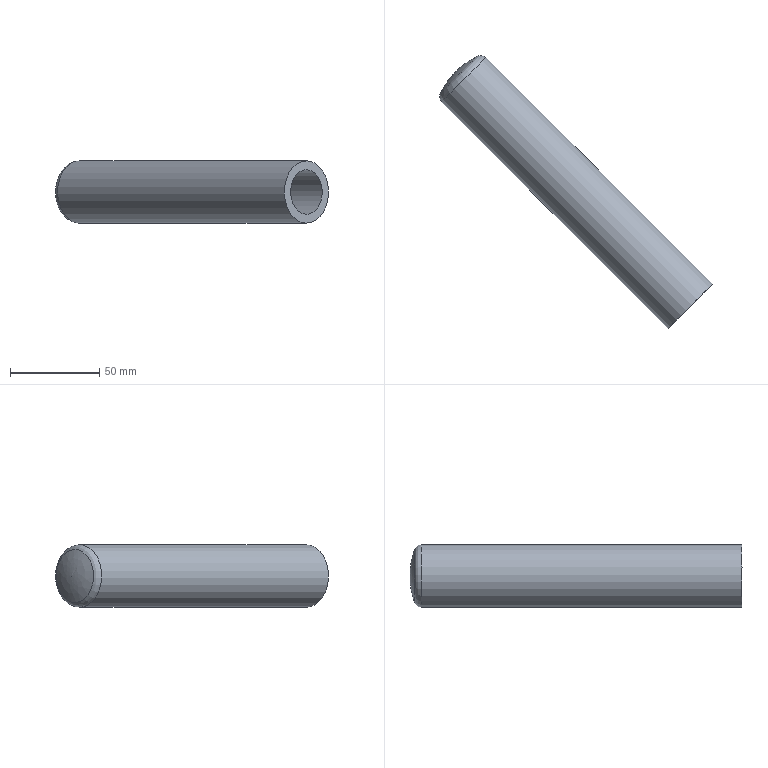Component | NX | GRIP_2 | 1 solid | 6 faces | box 152.97 x 152.97 x 35 mm | volume 88743 mm3 | cylinder 2 | plane 2 | spline 1 | torus 1 | commonest cylinder face diameters 35 x1 25 x1
STEP:
#1=CARTESIAN_POINT('',(0.,0.,0.));
#2=DIRECTION('',(0.,0.,1.));
#3=DIRECTION('',(1.,0.,0.));
#4=AXIS2_PLACEMENT_3D('',#1,#2,#3);
#5=CARTESIAN_POINT('',(-156.716,225.387,366.272));
#6=VERTEX_POINT('',#5);
#7=CARTESIAN_POINT('',(-164.39,217.713,380.));
#8=DIRECTION('',(0.7071,-0.7071,0.));
#9=DIRECTION('',(0.4386,0.4386,-0.7844));
#10=AXIS2_PLACEMENT_3D('',#7,#8,#9);
#11=CIRCLE('',#10,17.5);
#12=CARTESIAN_POINT('',(-164.616,217.938,380.));
#13=DIRECTION('',(0.7071,-0.7071,0.));
#14=DIRECTION('',(0.4386,0.4386,-0.7844));
#15=AXIS2_PLACEMENT_3D('',#12,#13,#14);
#16=CYLINDRICAL_SURFACE('',#15,17.5);
#17=CARTESIAN_POINT('',(0.,0.3185));
#18=DIRECTION('',(1.,-0.));
#19=VECTOR('',#18,1.);
#20=LINE('',#17,#19);
#21=(GEOMETRIC_REPRESENTATION_CONTEXT(2)PARAMETRIC_REPRESENTATION_CONTEXT()REPRESENTATION_CONTEXT('',''));
#22=DEFINITIONAL_REPRESENTATION('',(#20),#21);
#23=PCURVE('',#16,#22);
#24=CARTESIAN_POINT('',(-164.39,217.713,380.));
#25=DIRECTION('',(0.7071,-0.7071,0.));
#26=DIRECTION('',(0.4386,0.4386,-0.7844));
#27=AXIS2_PLACEMENT_3D('',#24,#25,#26);
#28=TOROIDAL_SURFACE('',#27,13.5,4.);
#29=CARTESIAN_POINT('',(0.,6.283));
#30=DIRECTION('',(1.,0.));
#31=VECTOR('',#30,1.);
#32=LINE('',#29,#31);
#33=(GEOMETRIC_REPRESENTATION_CONTEXT(2)PARAMETRIC_REPRESENTATION_CONTEXT()REPRESENTATION_CONTEXT('',''));
#34=DEFINITIONAL_REPRESENTATION('',(#32),#33);
#35=PCURVE('',#28,#34);
#36=SURFACE_CURVE('',#11,(#23,#35),.PCURVE_S1.);
#37=EDGE_CURVE('',#6,#6,#36,.T.);
#38=ORIENTED_EDGE('',*,*,#37,.T.);
#39=CARTESIAN_POINT('',(-29.662,98.333,366.272));
#40=VERTEX_POINT('',#39);
#41=CARTESIAN_POINT('',(-156.716,225.387,366.272));
#42=CARTESIAN_POINT('',(-29.662,98.333,366.272));
#43=B_SPLINE_CURVE_WITH_KNOTS('',1,(#41,#42),.UNSPECIFIED.,.F.,.F.,(2,2),(0.3185,180.),.PIECEWISE_BEZIER_KNOTS.);
#44=CARTESIAN_POINT('',(6.283,0.));
#45=DIRECTION('',(0.,1.));
#46=VECTOR('',#45,1.);
#47=LINE('',#44,#46);
#48=(GEOMETRIC_REPRESENTATION_CONTEXT(2)PARAMETRIC_REPRESENTATION_CONTEXT()REPRESENTATION_CONTEXT('',''));
#49=DEFINITIONAL_REPRESENTATION('',(#47),#48);
#50=PCURVE('',#16,#49);
#51=CARTESIAN_POINT('',(0.,0.));
#52=DIRECTION('',(0.,1.));
#53=VECTOR('',#52,1.);
#54=LINE('',#51,#53);
#55=(GEOMETRIC_REPRESENTATION_CONTEXT(2)PARAMETRIC_REPRESENTATION_CONTEXT()REPRESENTATION_CONTEXT('',''));
#56=DEFINITIONAL_REPRESENTATION('',(#54),#55);
#57=PCURVE('',#16,#56);
#58=SEAM_CURVE('',#43,(#50,#57),.PCURVE_S1.);
#59=EDGE_CURVE('',#6,#40,#58,.T.);
#60=ORIENTED_EDGE('',*,*,#59,.T.);
#61=CARTESIAN_POINT('',(-45.011,82.984,393.728));
#62=VERTEX_POINT('',#61);
#63=CARTESIAN_POINT('',(-37.336,90.659,380.));
#64=DIRECTION('',(0.7071,-0.7071,0.));
#65=DIRECTION('',(-0.4386,-0.4386,0.7844));
#66=AXIS2_PLACEMENT_3D('',#63,#64,#65);
#67=CIRCLE('',#66,17.5);
#68=CARTESIAN_POINT('',(3.142,180.));
#69=DIRECTION('',(1.,0.));
#70=VECTOR('',#69,1.);
#71=LINE('',#68,#70);
#72=(GEOMETRIC_REPRESENTATION_CONTEXT(2)PARAMETRIC_REPRESENTATION_CONTEXT()REPRESENTATION_CONTEXT('',''));
#73=DEFINITIONAL_REPRESENTATION('',(#71),#72);
#74=PCURVE('',#16,#73);
#75=CARTESIAN_POINT('',(-37.336,90.659,380.));
#76=DIRECTION('',(0.7071,-0.7071,0.));
#77=DIRECTION('',(0.4386,0.4386,-0.7844));
#78=AXIS2_PLACEMENT_3D('',#75,#76,#77);
#79=PLANE('',#78);
#80=CARTESIAN_POINT('',(0.,0.));
#81=DIRECTION('',(-1.,0.));
#82=AXIS2_PLACEMENT_2D('',#80,#81);
#83=CIRCLE('',#82,17.5);
#84=(GEOMETRIC_REPRESENTATION_CONTEXT(2)PARAMETRIC_REPRESENTATION_CONTEXT()REPRESENTATION_CONTEXT('',''));
#85=DEFINITIONAL_REPRESENTATION('',(#83),#84);
#86=PCURVE('',#79,#85);
#87=SURFACE_CURVE('',#67,(#74,#86),.PCURVE_S1.);
#88=EDGE_CURVE('',#62,#40,#87,.T.);
#89=ORIENTED_EDGE('',*,*,#88,.F.);
#90=CARTESIAN_POINT('',(-37.336,90.659,380.));
#91=DIRECTION('',(0.7071,-0.7071,0.));
#92=DIRECTION('',(-0.4386,-0.4386,0.7844));
#93=AXIS2_PLACEMENT_3D('',#90,#91,#92);
#94=CIRCLE('',#93,17.5);
#95=CARTESIAN_POINT('',(-3.142,180.));
#96=DIRECTION('',(1.,0.));
#97=VECTOR('',#96,1.);
#98=LINE('',#95,#97);
#99=(GEOMETRIC_REPRESENTATION_CONTEXT(2)PARAMETRIC_REPRESENTATION_CONTEXT()REPRESENTATION_CONTEXT('',''));
#100=DEFINITIONAL_REPRESENTATION('',(#98),#99);
#101=PCURVE('',#16,#100);
#102=CARTESIAN_POINT('',(0.,0.));
#103=DIRECTION('',(-1.,0.));
#104=AXIS2_PLACEMENT_2D('',#102,#103);
#105=CIRCLE('',#104,17.5);
#106=(GEOMETRIC_REPRESENTATION_CONTEXT(2)PARAMETRIC_REPRESENTATION_CONTEXT()REPRESENTATION_CONTEXT('',''));
#107=DEFINITIONAL_REPRESENTATION('',(#105),#106);
#108=PCURVE('',#79,#107);
#109=SURFACE_CURVE('',#94,(#101,#108),.PCURVE_S1.);
#110=EDGE_CURVE('',#40,#62,#109,.T.);
#111=ORIENTED_EDGE('',*,*,#110,.F.);
#112=ORIENTED_EDGE('',*,*,#59,.F.);
#113=EDGE_LOOP('',(#38,#60,#89,#111,#112));
#114=FACE_BOUND('',#113,.T.);
#115=ADVANCED_FACE('',(#114),#16,.T.);
#116=CARTESIAN_POINT('',(-170.097,212.456,389.805));
#117=VERTEX_POINT('',#116);
#118=CARTESIAN_POINT('',(-164.616,217.938,380.));
#119=DIRECTION('',(0.7071,-0.7071,0.));
#120=DIRECTION('',(-0.4386,-0.4386,0.7844));
#121=AXIS2_PLACEMENT_3D('',#118,#119,#120);
#122=CIRCLE('',#121,12.5);
#123=CARTESIAN_POINT('',(-164.616,217.938,380.));
#124=DIRECTION('',(0.7071,-0.7071,0.));
#125=DIRECTION('',(0.4386,0.4386,-0.7844));
#126=AXIS2_PLACEMENT_3D('',#123,#124,#125);
#127=CYLINDRICAL_SURFACE('',#126,12.5);
#128=CARTESIAN_POINT('',(3.142,0.));
#129=DIRECTION('',(1.,0.));
#130=VECTOR('',#129,1.);
#131=LINE('',#128,#130);
#132=(GEOMETRIC_REPRESENTATION_CONTEXT(2)PARAMETRIC_REPRESENTATION_CONTEXT()REPRESENTATION_CONTEXT('',''));
#133=DEFINITIONAL_REPRESENTATION('',(#131),#132);
#134=PCURVE('',#127,#133);
#135=CARTESIAN_POINT('',(-174.322,208.231,369.146));
#136=DIRECTION('',(0.7071,-0.7071,0.));
#137=DIRECTION('',(0.4386,0.4386,-0.7844));
#138=AXIS2_PLACEMENT_3D('',#135,#136,#137);
#139=PLANE('',#138);
#140=CARTESIAN_POINT('',(-0.,17.5));
#141=DIRECTION('',(-1.,-0.));
#142=AXIS2_PLACEMENT_2D('',#140,#141);
#143=CIRCLE('',#142,12.5);
#144=(GEOMETRIC_REPRESENTATION_CONTEXT(2)PARAMETRIC_REPRESENTATION_CONTEXT()REPRESENTATION_CONTEXT('',''));
#145=DEFINITIONAL_REPRESENTATION('',(#143),#144);
#146=PCURVE('',#139,#145);
#147=SURFACE_CURVE('',#122,(#134,#146),.PCURVE_S1.);
#148=EDGE_CURVE('',#117,#117,#147,.T.);
#149=ORIENTED_EDGE('',*,*,#148,.T.);
#150=CARTESIAN_POINT('',(-42.818,85.177,389.805));
#151=VERTEX_POINT('',#150);
#152=CARTESIAN_POINT('',(-170.097,212.456,389.805));
#153=CARTESIAN_POINT('',(-42.818,85.177,389.805));
#154=B_SPLINE_CURVE_WITH_KNOTS('',1,(#152,#153),.UNSPECIFIED.,.F.,.F.,(2,2),(0.,180.),.PIECEWISE_BEZIER_KNOTS.);
#155=CARTESIAN_POINT('',(9.425,0.));
#156=DIRECTION('',(0.,1.));
#157=VECTOR('',#156,1.);
#158=LINE('',#155,#157);
#159=(GEOMETRIC_REPRESENTATION_CONTEXT(2)PARAMETRIC_REPRESENTATION_CONTEXT()REPRESENTATION_CONTEXT('',''));
#160=DEFINITIONAL_REPRESENTATION('',(#158),#159);
#161=PCURVE('',#127,#160);
#162=CARTESIAN_POINT('',(3.142,0.));
#163=DIRECTION('',(0.,1.));
#164=VECTOR('',#163,1.);
#165=LINE('',#162,#164);
#166=(GEOMETRIC_REPRESENTATION_CONTEXT(2)PARAMETRIC_REPRESENTATION_CONTEXT()REPRESENTATION_CONTEXT('',''));
#167=DEFINITIONAL_REPRESENTATION('',(#165),#166);
#168=PCURVE('',#127,#167);
#169=SEAM_CURVE('',#154,(#161,#168),.PCURVE_S1.);
#170=EDGE_CURVE('',#117,#151,#169,.T.);
#171=ORIENTED_EDGE('',*,*,#170,.T.);
#172=CARTESIAN_POINT('',(-37.336,90.659,380.));
#173=DIRECTION('',(0.7071,-0.7071,0.));
#174=DIRECTION('',(-0.4386,-0.4386,0.7844));
#175=AXIS2_PLACEMENT_3D('',#172,#173,#174);
#176=CIRCLE('',#175,12.5);
#177=CARTESIAN_POINT('',(3.142,180.));
#178=DIRECTION('',(1.,0.));
#179=VECTOR('',#178,1.);
#180=LINE('',#177,#179);
#181=(GEOMETRIC_REPRESENTATION_CONTEXT(2)PARAMETRIC_REPRESENTATION_CONTEXT()REPRESENTATION_CONTEXT('',''));
#182=DEFINITIONAL_REPRESENTATION('',(#180),#181);
#183=PCURVE('',#127,#182);
#184=CARTESIAN_POINT('',(0.,0.));
#185=DIRECTION('',(-1.,-0.));
#186=AXIS2_PLACEMENT_2D('',#184,#185);
#187=CIRCLE('',#186,12.5);
#188=(GEOMETRIC_REPRESENTATION_CONTEXT(2)PARAMETRIC_REPRESENTATION_CONTEXT()REPRESENTATION_CONTEXT('',''));
#189=DEFINITIONAL_REPRESENTATION('',(#187),#188);
#190=PCURVE('',#79,#189);
#191=SURFACE_CURVE('',#176,(#183,#190),.PCURVE_S1.);
#192=EDGE_CURVE('',#151,#151,#191,.T.);
#193=ORIENTED_EDGE('',*,*,#192,.F.);
#194=ORIENTED_EDGE('',*,*,#170,.F.);
#195=EDGE_LOOP('',(#149,#171,#193,#194));
#196=FACE_BOUND('',#195,.F.);
#197=ADVANCED_FACE('',(#196),#127,.F.);
#198=ORIENTED_EDGE('',*,*,#88,.T.);
#199=ORIENTED_EDGE('',*,*,#110,.T.);
#200=EDGE_LOOP('',(#198,#199));
#201=FACE_BOUND('',#200,.T.);
#202=ORIENTED_EDGE('',*,*,#192,.F.);
#203=EDGE_LOOP('',(#202));
#204=FACE_BOUND('',#203,.T.);
#205=ADVANCED_FACE('',(#201,#204),#79,.T.);
#206=ORIENTED_EDGE('',*,*,#148,.T.);
#207=EDGE_LOOP('',(#206));
#208=FACE_BOUND('',#207,.T.);
#209=ADVANCED_FACE('',(#208),#139,.T.);
#210=CARTESIAN_POINT('',(-160.557,226.883,368.37));
#211=VERTEX_POINT('',#210);
#212=CARTESIAN_POINT('',(-173.561,213.879,391.63));
#213=VERTEX_POINT('',#212);
#214=CARTESIAN_POINT('',(-167.059,220.381,380.));
#215=DIRECTION('',(-0.7071,0.7071,0.));
#216=DIRECTION('',(0.4386,0.4386,-0.7844));
#217=AXIS2_PLACEMENT_3D('',#214,#215,#216);
#218=CIRCLE('',#217,14.826);
#219=CARTESIAN_POINT('',(-168.858,222.181,380.));
#220=CARTESIAN_POINT('',(-168.858,222.181,380.));
#221=CARTESIAN_POINT('',(-168.858,222.181,380.));
#222=CARTESIAN_POINT('',(-168.858,222.181,380.));
#223=CARTESIAN_POINT('',(-168.858,222.181,380.));
#224=CARTESIAN_POINT('',(-168.858,222.181,380.));
#225=CARTESIAN_POINT('',(-168.858,222.181,380.));
#226=CARTESIAN_POINT('',(-171.071,219.953,383.971));
#227=CARTESIAN_POINT('',(-165.455,225.569,390.249));
#228=CARTESIAN_POINT('',(-161.016,230.008,382.308));
#229=CARTESIAN_POINT('',(-166.631,224.393,376.029));
#230=CARTESIAN_POINT('',(-172.246,218.778,369.751));
#231=CARTESIAN_POINT('',(-176.686,214.338,377.692));
#232=CARTESIAN_POINT('',(-171.071,219.953,383.971));
#233=CARTESIAN_POINT('',(-172.653,217.16,387.884));
#234=CARTESIAN_POINT('',(-161.503,228.31,400.351));
#235=CARTESIAN_POINT('',(-152.688,237.125,384.583));
#236=CARTESIAN_POINT('',(-163.838,225.975,372.116));
#237=CARTESIAN_POINT('',(-174.987,214.826,359.649));
#238=CARTESIAN_POINT('',(-183.803,206.01,375.417));
#239=CARTESIAN_POINT('',(-172.653,217.16,387.884));
#240=CARTESIAN_POINT('',(-173.561,213.879,391.63));
#241=CARTESIAN_POINT('',(-157.113,230.327,410.021));
#242=CARTESIAN_POINT('',(-144.109,243.331,386.76));
#243=CARTESIAN_POINT('',(-160.557,226.883,368.37));
#244=CARTESIAN_POINT('',(-177.004,210.436,349.979));
#245=CARTESIAN_POINT('',(-190.008,197.432,373.24));
#246=CARTESIAN_POINT('',(-173.561,213.879,391.63));
#247=(BOUNDED_SURFACE()B_SPLINE_SURFACE(3,3,((#219,#220,#221,#222,#223,#224,#225),(#226,#227,#228,#229,#230,#231,#232),(#233,#234,#235,#236,#237,#238,#239),(#240,#241,#242,#243,#244,#245,#246)),.UNSPECIFIED.,.F.,.T.,.F.)B_SPLINE_SURFACE_WITH_KNOTS((4,4),(1,3,3,3,1),(0.,1.),(-0.5,0.,0.5,1.,1.5),.UNSPECIFIED.)GEOMETRIC_REPRESENTATION_ITEM()RATIONAL_B_SPLINE_SURFACE(((1.,0.3333,0.3333,1.,0.3333,0.3333,1.),(0.9906,0.3302,0.3302,0.9906,0.3302,0.3302,0.9906),(0.9906,0.3302,0.3302,0.9906,0.3302,0.3302,0.9906),(1.,0.3333,0.3333,1.,0.3333,0.3333,1.)))REPRESENTATION_ITEM('')SURFACE());
#248=CARTESIAN_POINT('',(1.,0.5));
#249=CARTESIAN_POINT('',(1.,0.5235));
#250=CARTESIAN_POINT('',(1.,0.5649));
#251=CARTESIAN_POINT('',(1.,0.6146));
#252=CARTESIAN_POINT('',(1.,0.6575));
#253=CARTESIAN_POINT('',(1.,0.696));
#254=CARTESIAN_POINT('',(1.,0.7322));
#255=CARTESIAN_POINT('',(1.,0.7678));
#256=CARTESIAN_POINT('',(1.,0.804));
#257=CARTESIAN_POINT('',(1.,0.8425));
#258=CARTESIAN_POINT('',(1.,0.8856));
#259=CARTESIAN_POINT('',(1.,0.9343));
#260=CARTESIAN_POINT('',(1.,1.));
#261=CARTESIAN_POINT('',(1.,1.066));
#262=CARTESIAN_POINT('',(1.,1.114));
#263=CARTESIAN_POINT('',(1.,1.158));
#264=CARTESIAN_POINT('',(1.,1.196));
#265=CARTESIAN_POINT('',(1.,1.232));
#266=CARTESIAN_POINT('',(1.,1.268));
#267=CARTESIAN_POINT('',(1.,1.304));
#268=CARTESIAN_POINT('',(1.,1.343));
#269=CARTESIAN_POINT('',(1.,1.385));
#270=CARTESIAN_POINT('',(1.,1.435));
#271=CARTESIAN_POINT('',(1.,1.476));
#272=CARTESIAN_POINT('',(1.,1.5));
#273=B_SPLINE_CURVE_WITH_KNOTS('',3,(#248,#249,#250,#251,#252,#253,#254,#255,#256,#257,#258,#259,#260,#261,#262,#263,#264,#265,#266,#267,#268,#269,#270,#271,#272),.UNSPECIFIED.,.F.,.F.,(4,1,1,1,1,1,1,1,1,1,1,1,1,1,1,1,1,1,1,1,1,1,4),(0.,0.2856,0.5712,0.8568,1.142,1.428,1.714,1.999,2.285,2.57,2.856,3.142,3.427,3.713,3.998,4.284,4.57,4.855,5.141,5.426,5.712,5.998,6.283),.QUASI_UNIFORM_KNOTS.);
#274=(GEOMETRIC_REPRESENTATION_CONTEXT(2)PARAMETRIC_REPRESENTATION_CONTEXT()REPRESENTATION_CONTEXT('',''));
#275=DEFINITIONAL_REPRESENTATION('',(#273),#274);
#276=PCURVE('',#247,#275);
#277=CARTESIAN_POINT('',(6.283,5.05));
#278=DIRECTION('',(-1.,0.));
#279=VECTOR('',#278,1.);
#280=LINE('',#277,#279);
#281=(GEOMETRIC_REPRESENTATION_CONTEXT(2)PARAMETRIC_REPRESENTATION_CONTEXT()REPRESENTATION_CONTEXT('',''));
#282=DEFINITIONAL_REPRESENTATION('',(#280),#281);
#283=PCURVE('',#28,#282);
#284=SURFACE_CURVE('',#218,(#276,#283),.PCURVE_S1.);
#285=EDGE_CURVE('',#211,#213,#284,.T.);
#286=ORIENTED_EDGE('',*,*,#285,.T.);
#287=CARTESIAN_POINT('',(-168.858,222.181,380.));
#288=VERTEX_POINT('',#287);
#289=CARTESIAN_POINT('',(-168.858,222.181,380.));
#290=CARTESIAN_POINT('',(-171.071,219.953,383.971));
#291=CARTESIAN_POINT('',(-172.653,217.16,387.884));
#292=CARTESIAN_POINT('',(-173.561,213.879,391.63));
#293=(BOUNDED_CURVE()B_SPLINE_CURVE(3,(#289,#290,#291,#292),.UNSPECIFIED.,.F.,.F.)B_SPLINE_CURVE_WITH_KNOTS((4,4),(0.,1.),.PIECEWISE_BEZIER_KNOTS.)CURVE()GEOMETRIC_REPRESENTATION_ITEM()RATIONAL_B_SPLINE_CURVE((1.,0.9906,0.9906,1.))REPRESENTATION_ITEM(''));
#294=CARTESIAN_POINT('',(0.,1.));
#295=DIRECTION('',(1.,0.));
#296=VECTOR('',#295,1.);
#297=LINE('',#294,#296);
#298=(GEOMETRIC_REPRESENTATION_CONTEXT(2)PARAMETRIC_REPRESENTATION_CONTEXT()REPRESENTATION_CONTEXT('',''));
#299=DEFINITIONAL_REPRESENTATION('',(#297),#298);
#300=PCURVE('',#247,#299);
#301=CARTESIAN_POINT('',(0.,0.));
#302=DIRECTION('',(1.,0.));
#303=VECTOR('',#302,1.);
#304=LINE('',#301,#303);
#305=(GEOMETRIC_REPRESENTATION_CONTEXT(2)PARAMETRIC_REPRESENTATION_CONTEXT()REPRESENTATION_CONTEXT('',''));
#306=DEFINITIONAL_REPRESENTATION('',(#304),#305);
#307=PCURVE('',#247,#306);
#308=SEAM_CURVE('',#293,(#300,#307),.PCURVE_S1.);
#309=EDGE_CURVE('',#288,#213,#308,.T.);
#310=ORIENTED_EDGE('',*,*,#309,.F.);
#311=ORIENTED_EDGE('',*,*,#309,.T.);
#312=CARTESIAN_POINT('',(-167.059,220.381,380.));
#313=DIRECTION('',(-0.7071,0.7071,0.));
#314=DIRECTION('',(0.4386,0.4386,-0.7844));
#315=AXIS2_PLACEMENT_3D('',#312,#313,#314);
#316=CIRCLE('',#315,14.826);
#317=CARTESIAN_POINT('',(1.,-0.5));
#318=CARTESIAN_POINT('',(1.,-0.4765));
#319=CARTESIAN_POINT('',(1.,-0.4351));
#320=CARTESIAN_POINT('',(1.,-0.3854));
#321=CARTESIAN_POINT('',(1.,-0.3425));
#322=CARTESIAN_POINT('',(1.,-0.304));
#323=CARTESIAN_POINT('',(1.,-0.2678));
#324=CARTESIAN_POINT('',(1.,-0.2322));
#325=CARTESIAN_POINT('',(1.,-0.196));
#326=CARTESIAN_POINT('',(1.,-0.1575));
#327=CARTESIAN_POINT('',(1.,-0.1144));
#328=CARTESIAN_POINT('',(1.,-0.06567));
#329=CARTESIAN_POINT('',(1.,-0.));
#330=CARTESIAN_POINT('',(1.,0.06567));
#331=CARTESIAN_POINT('',(1.,0.1144));
#332=CARTESIAN_POINT('',(1.,0.1575));
#333=CARTESIAN_POINT('',(1.,0.196));
#334=CARTESIAN_POINT('',(1.,0.2322));
#335=CARTESIAN_POINT('',(1.,0.2678));
#336=CARTESIAN_POINT('',(1.,0.304));
#337=CARTESIAN_POINT('',(1.,0.3425));
#338=CARTESIAN_POINT('',(1.,0.3854));
#339=CARTESIAN_POINT('',(1.,0.4351));
#340=CARTESIAN_POINT('',(1.,0.4765));
#341=CARTESIAN_POINT('',(1.,0.5));
#342=B_SPLINE_CURVE_WITH_KNOTS('',3,(#317,#318,#319,#320,#321,#322,#323,#324,#325,#326,#327,#328,#329,#330,#331,#332,#333,#334,#335,#336,#337,#338,#339,#340,#341),.UNSPECIFIED.,.F.,.F.,(4,1,1,1,1,1,1,1,1,1,1,1,1,1,1,1,1,1,1,1,1,1,4),(0.,0.2856,0.5712,0.8568,1.142,1.428,1.714,1.999,2.285,2.57,2.856,3.142,3.427,3.713,3.998,4.284,4.57,4.855,5.141,5.426,5.712,5.998,6.283),.QUASI_UNIFORM_KNOTS.);
#343=(GEOMETRIC_REPRESENTATION_CONTEXT(2)PARAMETRIC_REPRESENTATION_CONTEXT()REPRESENTATION_CONTEXT('',''));
#344=DEFINITIONAL_REPRESENTATION('',(#342),#343);
#345=PCURVE('',#247,#344);
#346=CARTESIAN_POINT('',(6.283,5.05));
#347=DIRECTION('',(-1.,-0.));
#348=VECTOR('',#347,1.);
#349=LINE('',#346,#348);
#350=(GEOMETRIC_REPRESENTATION_CONTEXT(2)PARAMETRIC_REPRESENTATION_CONTEXT()REPRESENTATION_CONTEXT('',''));
#351=DEFINITIONAL_REPRESENTATION('',(#349),#350);
#352=PCURVE('',#28,#351);
#353=SURFACE_CURVE('',#316,(#345,#352),.PCURVE_S1.);
#354=EDGE_CURVE('',#213,#211,#353,.T.);
#355=ORIENTED_EDGE('',*,*,#354,.T.);
#356=EDGE_LOOP('',(#286,#310,#311,#355));
#357=FACE_BOUND('',#356,.T.);
#358=ADVANCED_FACE('',(#357),#247,.T.);
#359=ORIENTED_EDGE('',*,*,#37,.F.);
#360=CARTESIAN_POINT('',(-160.557,226.883,368.37));
#361=CARTESIAN_POINT('',(-160.017,227.032,367.754));
#362=CARTESIAN_POINT('',(-159.378,227.011,367.201));
#363=CARTESIAN_POINT('',(-158.682,226.818,366.751));
#364=CARTESIAN_POINT('',(-157.974,226.465,366.435));
#365=CARTESIAN_POINT('',(-157.304,225.976,366.272));
#366=CARTESIAN_POINT('',(-156.716,225.387,366.272));
#367=(BOUNDED_CURVE()B_SPLINE_CURVE(6,(#360,#361,#362,#363,#364,#365,#366),.UNSPECIFIED.,.F.,.F.)B_SPLINE_CURVE_WITH_KNOTS((7,7),(-1.233,0.),.PIECEWISE_BEZIER_KNOTS.)CURVE()GEOMETRIC_REPRESENTATION_ITEM()RATIONAL_B_SPLINE_CURVE((1.019,1.006,0.9987,0.9963,0.9987,1.006,1.019))REPRESENTATION_ITEM(''));
#368=CARTESIAN_POINT('',(0.,6.283));
#369=DIRECTION('',(0.,1.));
#370=VECTOR('',#369,1.);
#371=LINE('',#368,#370);
#372=(GEOMETRIC_REPRESENTATION_CONTEXT(2)PARAMETRIC_REPRESENTATION_CONTEXT()REPRESENTATION_CONTEXT('',''));
#373=DEFINITIONAL_REPRESENTATION('',(#371),#372);
#374=PCURVE('',#28,#373);
#375=CARTESIAN_POINT('',(6.283,6.283));
#376=DIRECTION('',(0.,1.));
#377=VECTOR('',#376,1.);
#378=LINE('',#375,#377);
#379=(GEOMETRIC_REPRESENTATION_CONTEXT(2)PARAMETRIC_REPRESENTATION_CONTEXT()REPRESENTATION_CONTEXT('',''));
#380=DEFINITIONAL_REPRESENTATION('',(#378),#379);
#381=PCURVE('',#28,#380);
#382=SEAM_CURVE('',#367,(#374,#381),.PCURVE_S1.);
#383=EDGE_CURVE('',#211,#6,#382,.T.);
#384=ORIENTED_EDGE('',*,*,#383,.F.);
#385=ORIENTED_EDGE('',*,*,#354,.F.);
#386=ORIENTED_EDGE('',*,*,#285,.F.);
#387=ORIENTED_EDGE('',*,*,#383,.T.);
#388=EDGE_LOOP('',(#359,#384,#385,#386,#387));
#389=FACE_BOUND('',#388,.T.);
#390=ADVANCED_FACE('',(#389),#28,.T.);
#391=CLOSED_SHELL('',(#115,#197,#205,#209,#358,#390));
#392=MANIFOLD_SOLID_BREP('',#391);
#393=(LENGTH_UNIT()NAMED_UNIT(*)SI_UNIT(.MILLI.,.METRE.));
#394=UNCERTAINTY_MEASURE_WITH_UNIT(LENGTH_MEASURE(0.01),#393,'','');
#395=(NAMED_UNIT(*)PLANE_ANGLE_UNIT()SI_UNIT($,.RADIAN.));
#396=(NAMED_UNIT(*)SI_UNIT($,.STERADIAN.)SOLID_ANGLE_UNIT());
#397=(GEOMETRIC_REPRESENTATION_CONTEXT(3)GLOBAL_UNCERTAINTY_ASSIGNED_CONTEXT((#394))GLOBAL_UNIT_ASSIGNED_CONTEXT((#393,#395,#396))REPRESENTATION_CONTEXT('',''));
#398=ADVANCED_BREP_SHAPE_REPRESENTATION('',(#4,#392),#397);